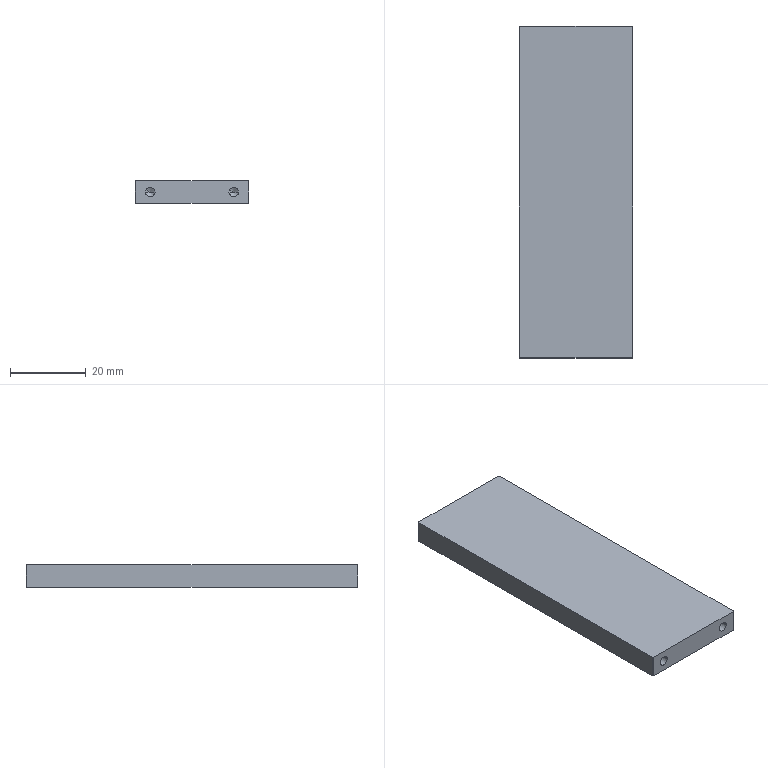CAM job | Mastercam | mm | 15 operations | part box 30 x 87.5 x 6
1. Facing | 1 - D80-R0.8 J-面铣刀
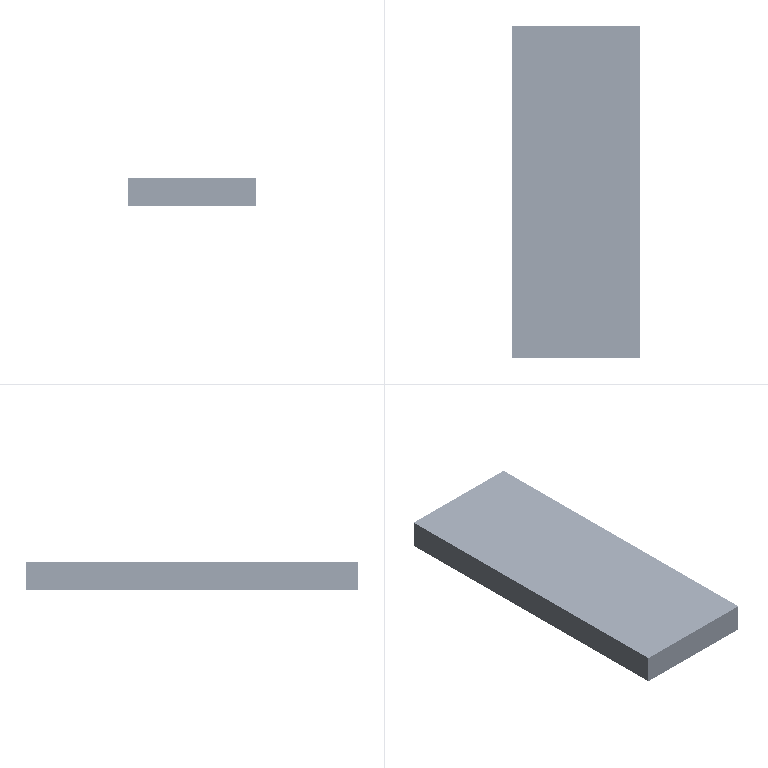2. 2D High Speed (2D Dynamic Mill) | 9 - D10-C 平底刀
3. Facing | 1 - D80-R0.8 J-面铣刀
4. Contour (2D) | 10 - D10-J 平底刀
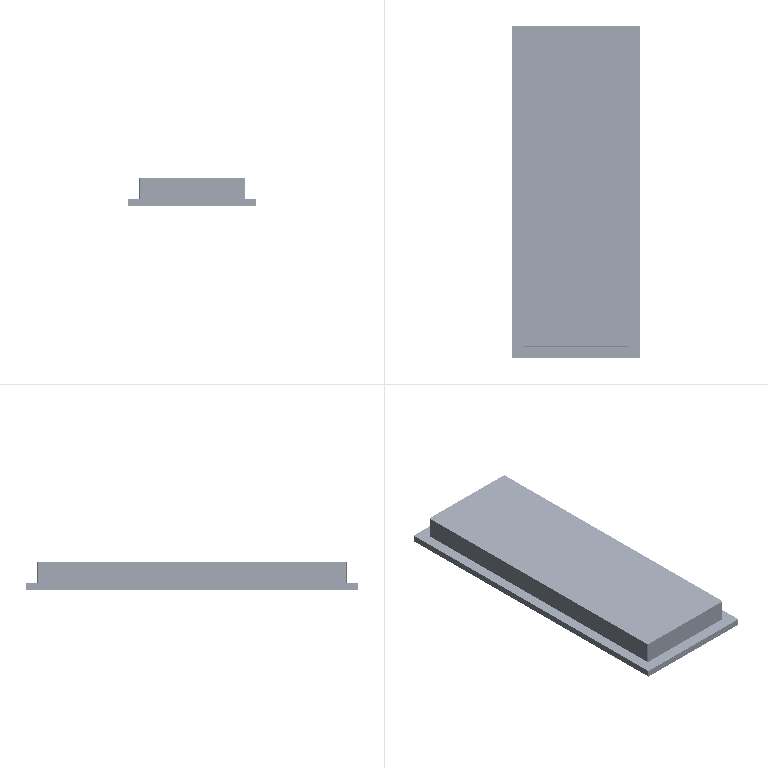5. Model Chamfer | 2 - D6定心倒角刀
6. Drill/Counterbore | 2 - D6定心倒角刀
7. Peck Drill | 16 - 2.5 钻头
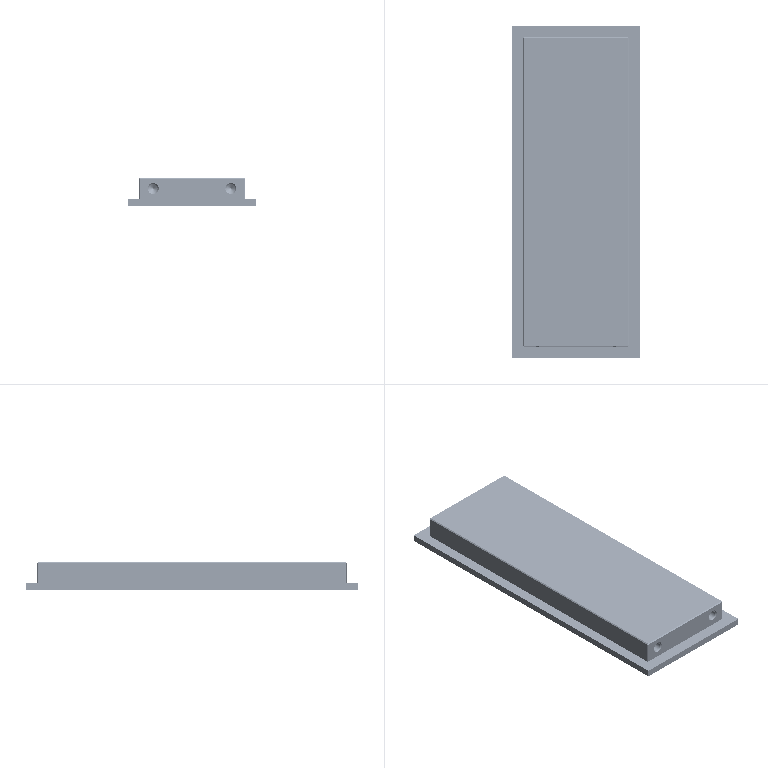8. Chamfer Drill | 2 - D6定心倒角刀
9. Thread Mill | 22 - M3/0.5  -D2.4L9螺纹铣刀
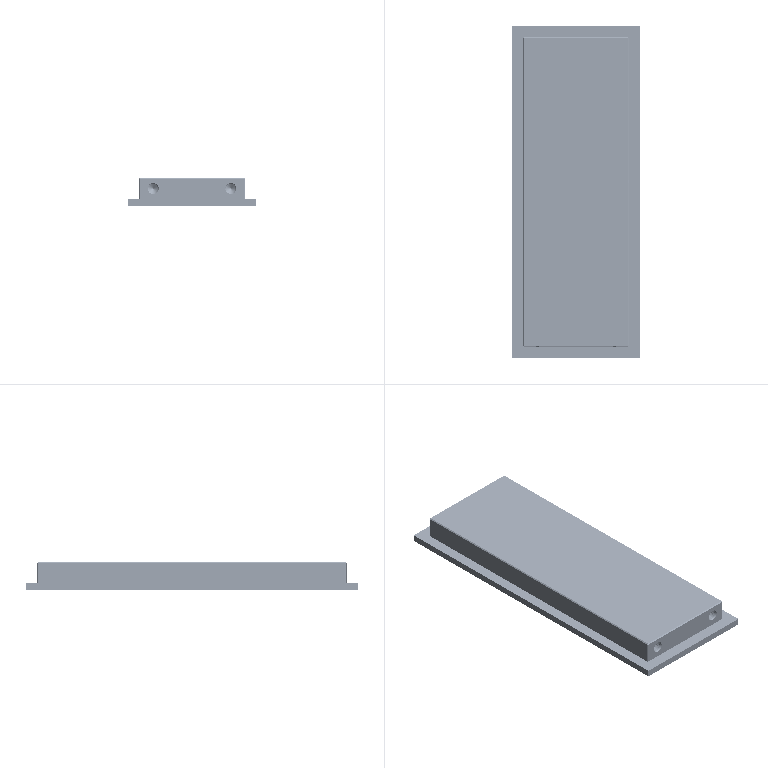10. Drill/Counterbore | 2 - D6定心倒角刀
11. Peck Drill | 16 - 2.5 钻头
12. Chamfer Drill | 2 - D6定心倒角刀
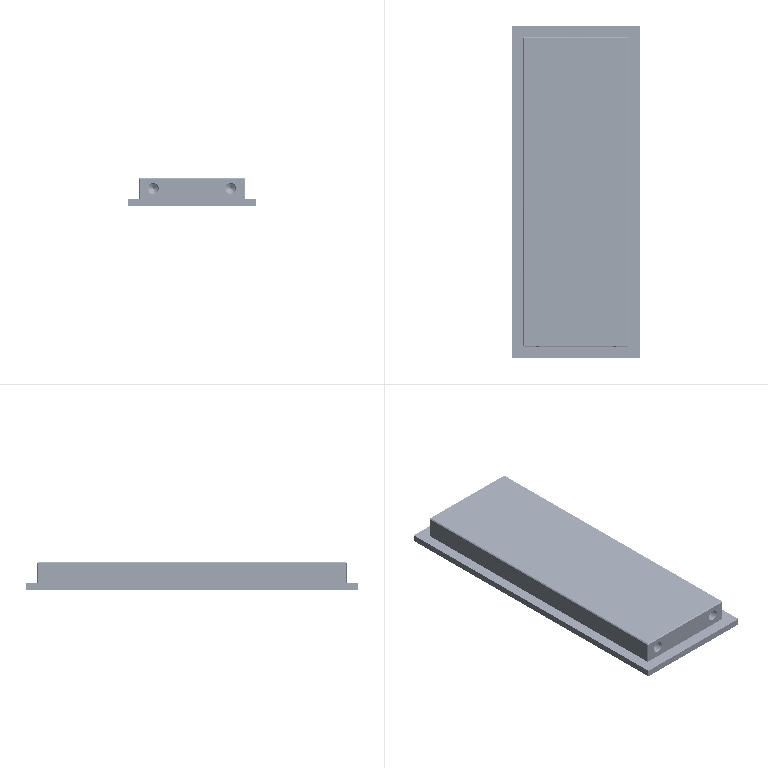13. Thread Mill | 22 - M3/0.5  -D2.4L9螺纹铣刀
14. Facing | 1 - D80-R0.8 J-面铣刀
15. Model Chamfer | 2 - D6定心倒角刀